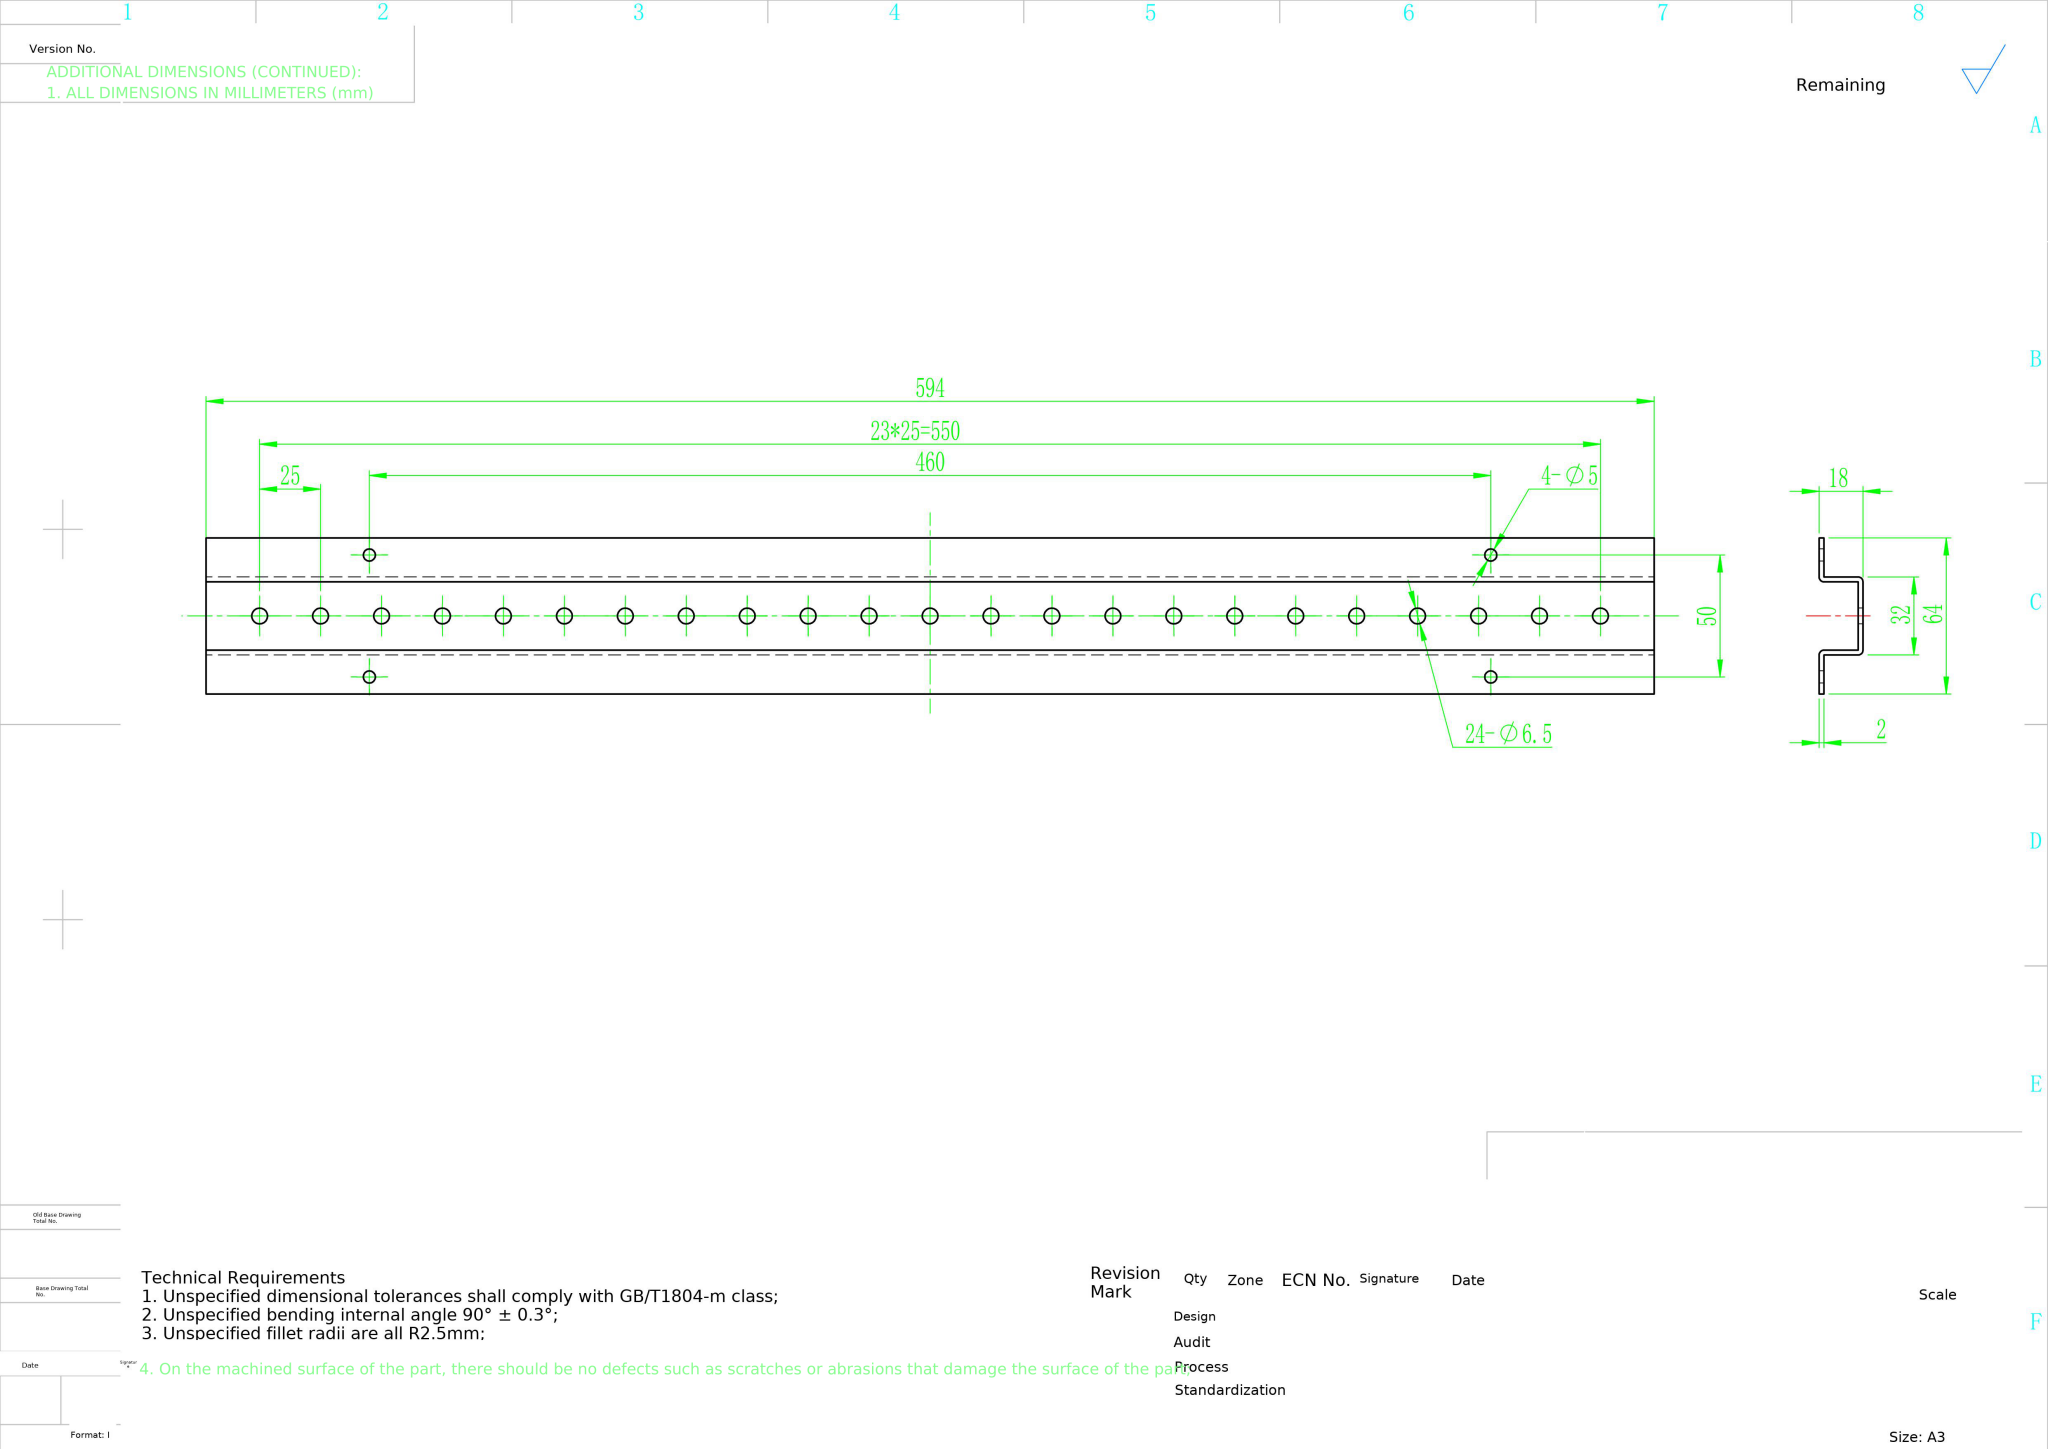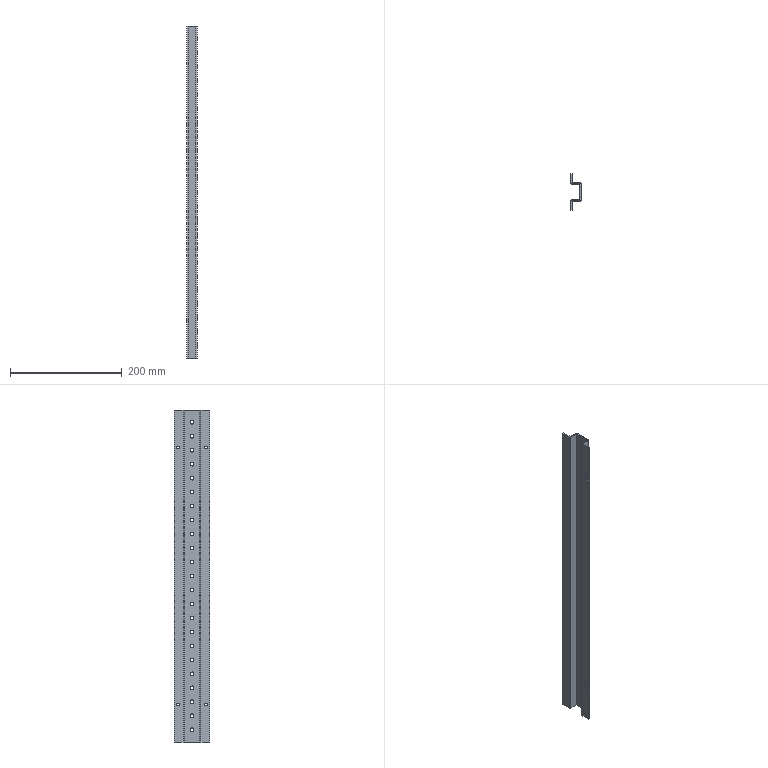Part | NX | mm | 1 solid | 92 faces | box 18 x 64 x 594 mm | volume 110323 mm3 | cylinder 62 | plane 30 | commonest cylinder face diameters 6.5 x46 5 x8 4.002 x4 0.002 x4